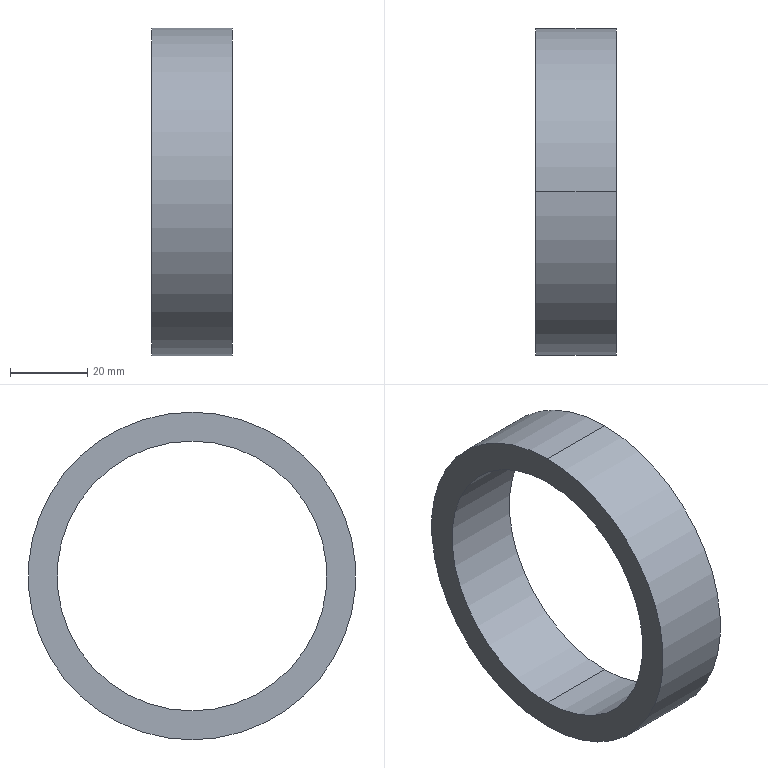Component | SolidWorks | bearing dan rumahan assembly-1_penahan bearing-1 | 1 solid | 6 faces | box 21 x 85 x 85 mm | volume 38347 mm3 | cylinder 4 | plane 2 | commonest cylinder face diameters 70 x2 85 x2
build123d program:
from build123d import *

# Parameters (mm, degrees)
SKETCH2_R           = 42.5
SKETCH2_R_2         = 35
BOSS_EXTRUDE1_DEPTH = 21


with BuildPart() as part:
    # Sketch2 → Boss-Extrude1 (new body)
    with BuildSketch(Plane(origin=(0, 0, 0), x_dir=(0, 0, -1), z_dir=(1, 0, 0))):
        with Locations(Location((0, 0, 0), (0, 0, 180))):
            Circle(SKETCH2_R)
        with Locations(Location((0, 0, 0), (0, 0, 180))):
            Circle(SKETCH2_R_2, mode=Mode.SUBTRACT)
    extrude(amount=BOSS_EXTRUDE1_DEPTH)


solid = part.part

# Placed as in the assembly
solid = solid.moved(Location((16.5, -110, 40), (0, 0, 0)))
STEP:
#1=COLOUR_RGB('',0.7922,0.8196,0.9333);
#2=FILL_AREA_STYLE_COLOUR('',#1);
#3=FILL_AREA_STYLE('',(#2));
#4=SURFACE_STYLE_FILL_AREA(#3);
#5=SURFACE_SIDE_STYLE('',(#4));
#6=SURFACE_STYLE_USAGE(.BOTH.,#5);
#7=PRESENTATION_STYLE_ASSIGNMENT((#6));
#8=CARTESIAN_POINT('',(1.476,-4.331,2.953));
#9=VERTEX_POINT('',#8);
#10=CARTESIAN_POINT('',(1.476,-4.331,0.1969));
#11=VERTEX_POINT('',#10);
#12=CARTESIAN_POINT('',(1.476,-4.331,1.575));
#13=DIRECTION('',(1.,0.,0.));
#14=DIRECTION('',(0.,0.,-1.));
#15=AXIS2_PLACEMENT_3D('',#12,#13,#14);
#16=CIRCLE('',#15,1.378);
#17=EDGE_CURVE('',#9,#11,#16,.T.);
#18=ORIENTED_EDGE('',*,*,#17,.T.);
#19=CARTESIAN_POINT('',(0.6496,-4.331,0.1969));
#20=VERTEX_POINT('',#19);
#21=CARTESIAN_POINT('',(1.476,-4.331,0.1969));
#22=DIRECTION('',(-1.,0.,0.));
#23=VECTOR('',#22,39.37);
#24=LINE('',#21,#23);
#25=EDGE_CURVE('',#11,#20,#24,.T.);
#26=ORIENTED_EDGE('',*,*,#25,.T.);
#27=CARTESIAN_POINT('',(0.6496,-4.331,2.953));
#28=VERTEX_POINT('',#27);
#29=CARTESIAN_POINT('',(0.6496,-4.331,1.575));
#30=DIRECTION('',(1.,0.,0.));
#31=DIRECTION('',(0.,0.,-1.));
#32=AXIS2_PLACEMENT_3D('',#29,#30,#31);
#33=CIRCLE('',#32,1.378);
#34=EDGE_CURVE('',#28,#20,#33,.T.);
#35=ORIENTED_EDGE('',*,*,#34,.F.);
#36=CARTESIAN_POINT('',(1.476,-4.331,2.953));
#37=DIRECTION('',(-1.,0.,0.));
#38=VECTOR('',#37,39.37);
#39=LINE('',#36,#38);
#40=EDGE_CURVE('',#9,#28,#39,.T.);
#41=ORIENTED_EDGE('',*,*,#40,.F.);
#42=EDGE_LOOP('',(#18,#26,#35,#41));
#43=FACE_OUTER_BOUND('',#42,.T.);
#44=CARTESIAN_POINT('',(1.476,-4.331,1.575));
#45=DIRECTION('',(-1.,0.,0.));
#46=DIRECTION('',(0.,0.,1.));
#47=AXIS2_PLACEMENT_3D('',#44,#45,#46);
#48=CYLINDRICAL_SURFACE('',#47,1.378);
#49=ADVANCED_FACE('',(#43),#48,.F.);
#50=CARTESIAN_POINT('',(1.476,-4.331,-0.09843));
#51=VERTEX_POINT('',#50);
#52=CARTESIAN_POINT('',(1.476,-4.331,3.248));
#53=VERTEX_POINT('',#52);
#54=CARTESIAN_POINT('',(1.476,-4.331,1.575));
#55=DIRECTION('',(1.,0.,0.));
#56=DIRECTION('',(0.,0.,-1.));
#57=AXIS2_PLACEMENT_3D('',#54,#55,#56);
#58=CIRCLE('',#57,1.673);
#59=EDGE_CURVE('',#51,#53,#58,.T.);
#60=ORIENTED_EDGE('',*,*,#59,.F.);
#61=CARTESIAN_POINT('',(0.6496,-4.331,-0.09843));
#62=VERTEX_POINT('',#61);
#63=CARTESIAN_POINT('',(1.476,-4.331,-0.09843));
#64=DIRECTION('',(-1.,0.,0.));
#65=VECTOR('',#64,39.37);
#66=LINE('',#63,#65);
#67=EDGE_CURVE('',#51,#62,#66,.T.);
#68=ORIENTED_EDGE('',*,*,#67,.T.);
#69=CARTESIAN_POINT('',(0.6496,-4.331,3.248));
#70=VERTEX_POINT('',#69);
#71=CARTESIAN_POINT('',(0.6496,-4.331,1.575));
#72=DIRECTION('',(1.,0.,0.));
#73=DIRECTION('',(0.,0.,-1.));
#74=AXIS2_PLACEMENT_3D('',#71,#72,#73);
#75=CIRCLE('',#74,1.673);
#76=EDGE_CURVE('',#62,#70,#75,.T.);
#77=ORIENTED_EDGE('',*,*,#76,.T.);
#78=CARTESIAN_POINT('',(1.476,-4.331,3.248));
#79=DIRECTION('',(-1.,0.,0.));
#80=VECTOR('',#79,39.37);
#81=LINE('',#78,#80);
#82=EDGE_CURVE('',#53,#70,#81,.T.);
#83=ORIENTED_EDGE('',*,*,#82,.F.);
#84=EDGE_LOOP('',(#60,#68,#77,#83));
#85=FACE_OUTER_BOUND('',#84,.T.);
#86=CARTESIAN_POINT('',(1.476,-4.331,1.575));
#87=DIRECTION('',(-1.,0.,0.));
#88=DIRECTION('',(0.,0.,1.));
#89=AXIS2_PLACEMENT_3D('',#86,#87,#88);
#90=CYLINDRICAL_SURFACE('',#89,1.673);
#91=ADVANCED_FACE('',(#85),#90,.T.);
#92=CARTESIAN_POINT('',(1.476,-4.331,1.575));
#93=DIRECTION('',(1.,0.,0.));
#94=DIRECTION('',(0.,0.,-1.));
#95=AXIS2_PLACEMENT_3D('',#92,#93,#94);
#96=CIRCLE('',#95,1.673);
#97=EDGE_CURVE('',#53,#51,#96,.T.);
#98=ORIENTED_EDGE('',*,*,#97,.T.);
#99=ORIENTED_EDGE('',*,*,#59,.T.);
#100=EDGE_LOOP('',(#98,#99));
#101=FACE_OUTER_BOUND('',#100,.T.);
#102=ORIENTED_EDGE('',*,*,#17,.F.);
#103=CARTESIAN_POINT('',(1.476,-4.331,1.575));
#104=DIRECTION('',(1.,0.,0.));
#105=DIRECTION('',(0.,0.,-1.));
#106=AXIS2_PLACEMENT_3D('',#103,#104,#105);
#107=CIRCLE('',#106,1.378);
#108=EDGE_CURVE('',#11,#9,#107,.T.);
#109=ORIENTED_EDGE('',*,*,#108,.F.);
#110=EDGE_LOOP('',(#102,#109));
#111=FACE_BOUND('',#110,.T.);
#112=CARTESIAN_POINT('',(1.476,-4.331,1.575));
#113=DIRECTION('',(1.,0.,0.));
#114=DIRECTION('',(0.,0.,-1.));
#115=AXIS2_PLACEMENT_3D('',#112,#113,#114);
#116=PLANE('',#115);
#117=ADVANCED_FACE('',(#101,#111),#116,.T.);
#118=CARTESIAN_POINT('',(0.6496,-4.331,1.575));
#119=DIRECTION('',(1.,0.,0.));
#120=DIRECTION('',(0.,0.,-1.));
#121=AXIS2_PLACEMENT_3D('',#118,#119,#120);
#122=CIRCLE('',#121,1.673);
#123=EDGE_CURVE('',#70,#62,#122,.T.);
#124=ORIENTED_EDGE('',*,*,#123,.F.);
#125=ORIENTED_EDGE('',*,*,#76,.F.);
#126=EDGE_LOOP('',(#124,#125));
#127=FACE_OUTER_BOUND('',#126,.T.);
#128=ORIENTED_EDGE('',*,*,#34,.T.);
#129=CARTESIAN_POINT('',(0.6496,-4.331,1.575));
#130=DIRECTION('',(1.,0.,0.));
#131=DIRECTION('',(0.,0.,-1.));
#132=AXIS2_PLACEMENT_3D('',#129,#130,#131);
#133=CIRCLE('',#132,1.378);
#134=EDGE_CURVE('',#20,#28,#133,.T.);
#135=ORIENTED_EDGE('',*,*,#134,.T.);
#136=EDGE_LOOP('',(#128,#135));
#137=FACE_BOUND('',#136,.T.);
#138=CARTESIAN_POINT('',(0.6496,-4.331,1.575));
#139=DIRECTION('',(1.,0.,0.));
#140=DIRECTION('',(0.,0.,-1.));
#141=AXIS2_PLACEMENT_3D('',#138,#139,#140);
#142=PLANE('',#141);
#143=ADVANCED_FACE('',(#127,#137),#142,.F.);
#144=ORIENTED_EDGE('',*,*,#67,.F.);
#145=ORIENTED_EDGE('',*,*,#97,.F.);
#146=ORIENTED_EDGE('',*,*,#82,.T.);
#147=ORIENTED_EDGE('',*,*,#123,.T.);
#148=EDGE_LOOP('',(#144,#145,#146,#147));
#149=FACE_OUTER_BOUND('',#148,.T.);
#150=CARTESIAN_POINT('',(1.476,-4.331,1.575));
#151=DIRECTION('',(-1.,0.,0.));
#152=DIRECTION('',(0.,0.,1.));
#153=AXIS2_PLACEMENT_3D('',#150,#151,#152);
#154=CYLINDRICAL_SURFACE('',#153,1.673);
#155=ADVANCED_FACE('',(#149),#154,.T.);
#156=ORIENTED_EDGE('',*,*,#25,.F.);
#157=ORIENTED_EDGE('',*,*,#108,.T.);
#158=ORIENTED_EDGE('',*,*,#40,.T.);
#159=ORIENTED_EDGE('',*,*,#134,.F.);
#160=EDGE_LOOP('',(#156,#157,#158,#159));
#161=FACE_OUTER_BOUND('',#160,.T.);
#162=CARTESIAN_POINT('',(1.476,-4.331,1.575));
#163=DIRECTION('',(-1.,0.,0.));
#164=DIRECTION('',(0.,0.,1.));
#165=AXIS2_PLACEMENT_3D('',#162,#163,#164);
#166=CYLINDRICAL_SURFACE('',#165,1.378);
#167=ADVANCED_FACE('',(#161),#166,.F.);
#168=CLOSED_SHELL('',(#49,#91,#117,#143,#155,#167));
#169=MANIFOLD_SOLID_BREP('',#168);
#170=STYLED_ITEM('',(#7),#169);
#171=PRESENTATION_LAYER_ASSIGNMENT('','',(#170));
#172=(LENGTH_UNIT()NAMED_UNIT(*)SI_UNIT($,.METRE.));
#173=LENGTH_MEASURE_WITH_UNIT(LENGTH_MEASURE(0.0254),#172);
#174=DIMENSIONAL_EXPONENTS(1.,0.,0.,0.,0.,0.,0.);
#175=(CONVERSION_BASED_UNIT('',#173)LENGTH_UNIT()NAMED_UNIT(#174));
#176=UNCERTAINTY_MEASURE_WITH_UNIT(LENGTH_MEASURE(0.00001),#175,'','');
#177=(NAMED_UNIT(*)PLANE_ANGLE_UNIT()SI_UNIT($,.RADIAN.));
#178=(NAMED_UNIT(*)SI_UNIT($,.STERADIAN.)SOLID_ANGLE_UNIT());
#179=(GEOMETRIC_REPRESENTATION_CONTEXT(3)GLOBAL_UNCERTAINTY_ASSIGNED_CONTEXT((#176))GLOBAL_UNIT_ASSIGNED_CONTEXT((#175,#177,#178))REPRESENTATION_CONTEXT('',''));
#180=MECHANICAL_DESIGN_GEOMETRIC_PRESENTATION_REPRESENTATION('',(#170),#179);
#181=CARTESIAN_POINT('',(0.,0.,0.));
#182=DIRECTION('',(0.,0.,1.));
#183=DIRECTION('',(1.,0.,0.));
#184=AXIS2_PLACEMENT_3D('',#181,#182,#183);
#185=(LENGTH_UNIT()NAMED_UNIT(*)SI_UNIT($,.METRE.));
#186=LENGTH_MEASURE_WITH_UNIT(LENGTH_MEASURE(0.0254),#185);
#187=DIMENSIONAL_EXPONENTS(1.,0.,0.,0.,0.,0.,0.);
#188=(CONVERSION_BASED_UNIT('',#186)LENGTH_UNIT()NAMED_UNIT(#187));
#189=UNCERTAINTY_MEASURE_WITH_UNIT(LENGTH_MEASURE(0.00001),#188,'','');
#190=(NAMED_UNIT(*)PLANE_ANGLE_UNIT()SI_UNIT($,.RADIAN.));
#191=(NAMED_UNIT(*)SI_UNIT($,.STERADIAN.)SOLID_ANGLE_UNIT());
#192=(GEOMETRIC_REPRESENTATION_CONTEXT(3)GLOBAL_UNCERTAINTY_ASSIGNED_CONTEXT((#189))GLOBAL_UNIT_ASSIGNED_CONTEXT((#188,#190,#191))REPRESENTATION_CONTEXT('',''));
#193=ADVANCED_BREP_SHAPE_REPRESENTATION('',(#169,#184),#192);